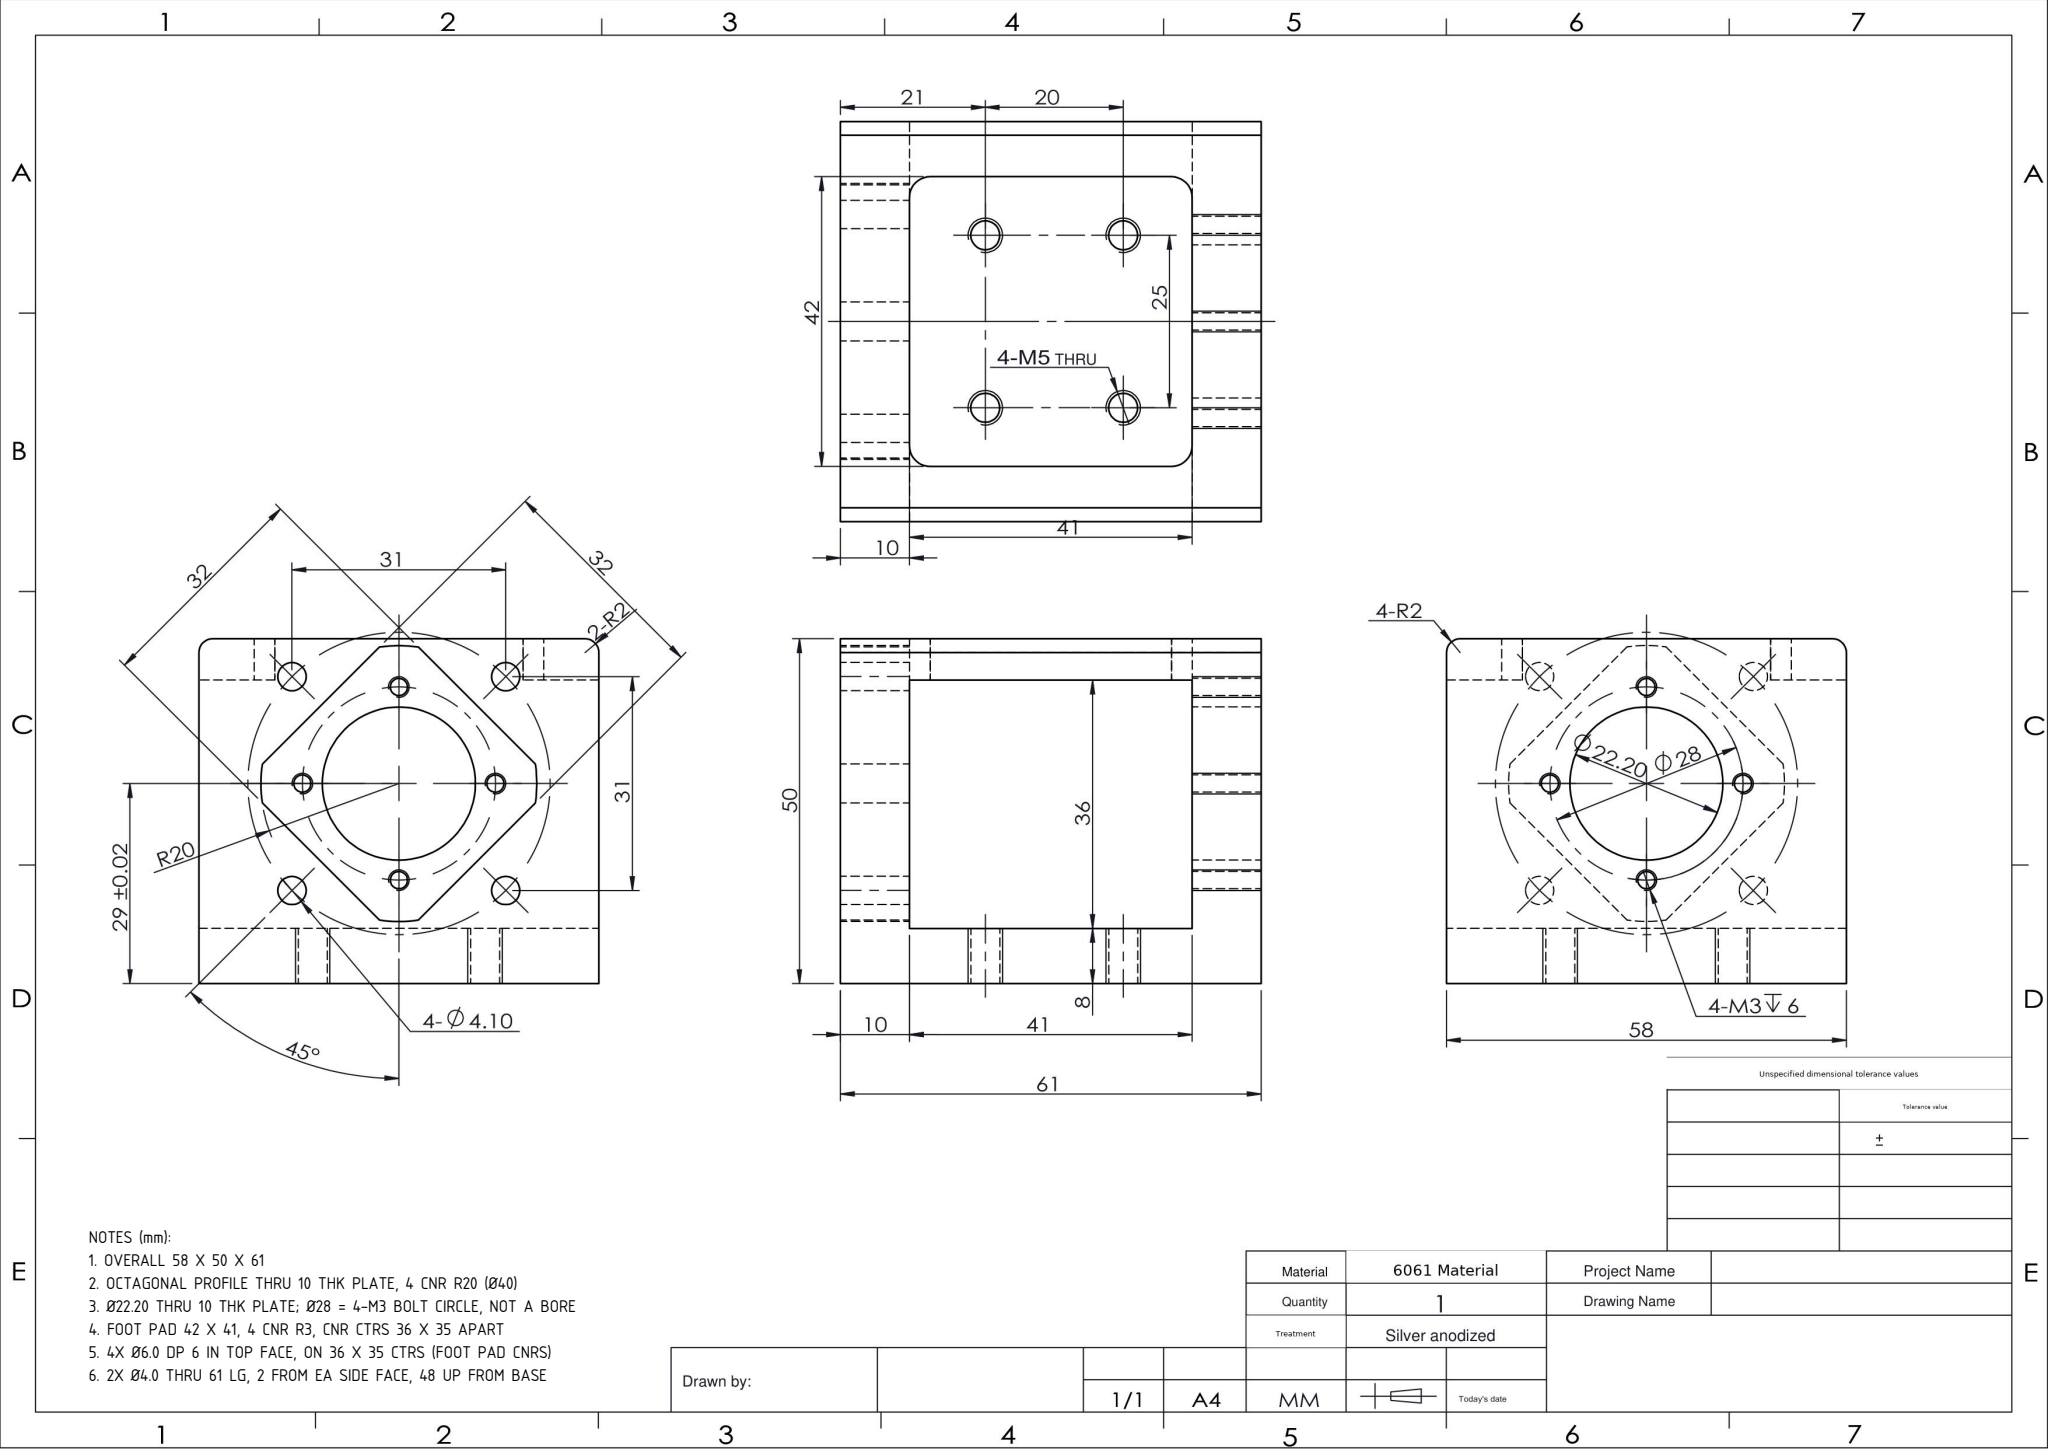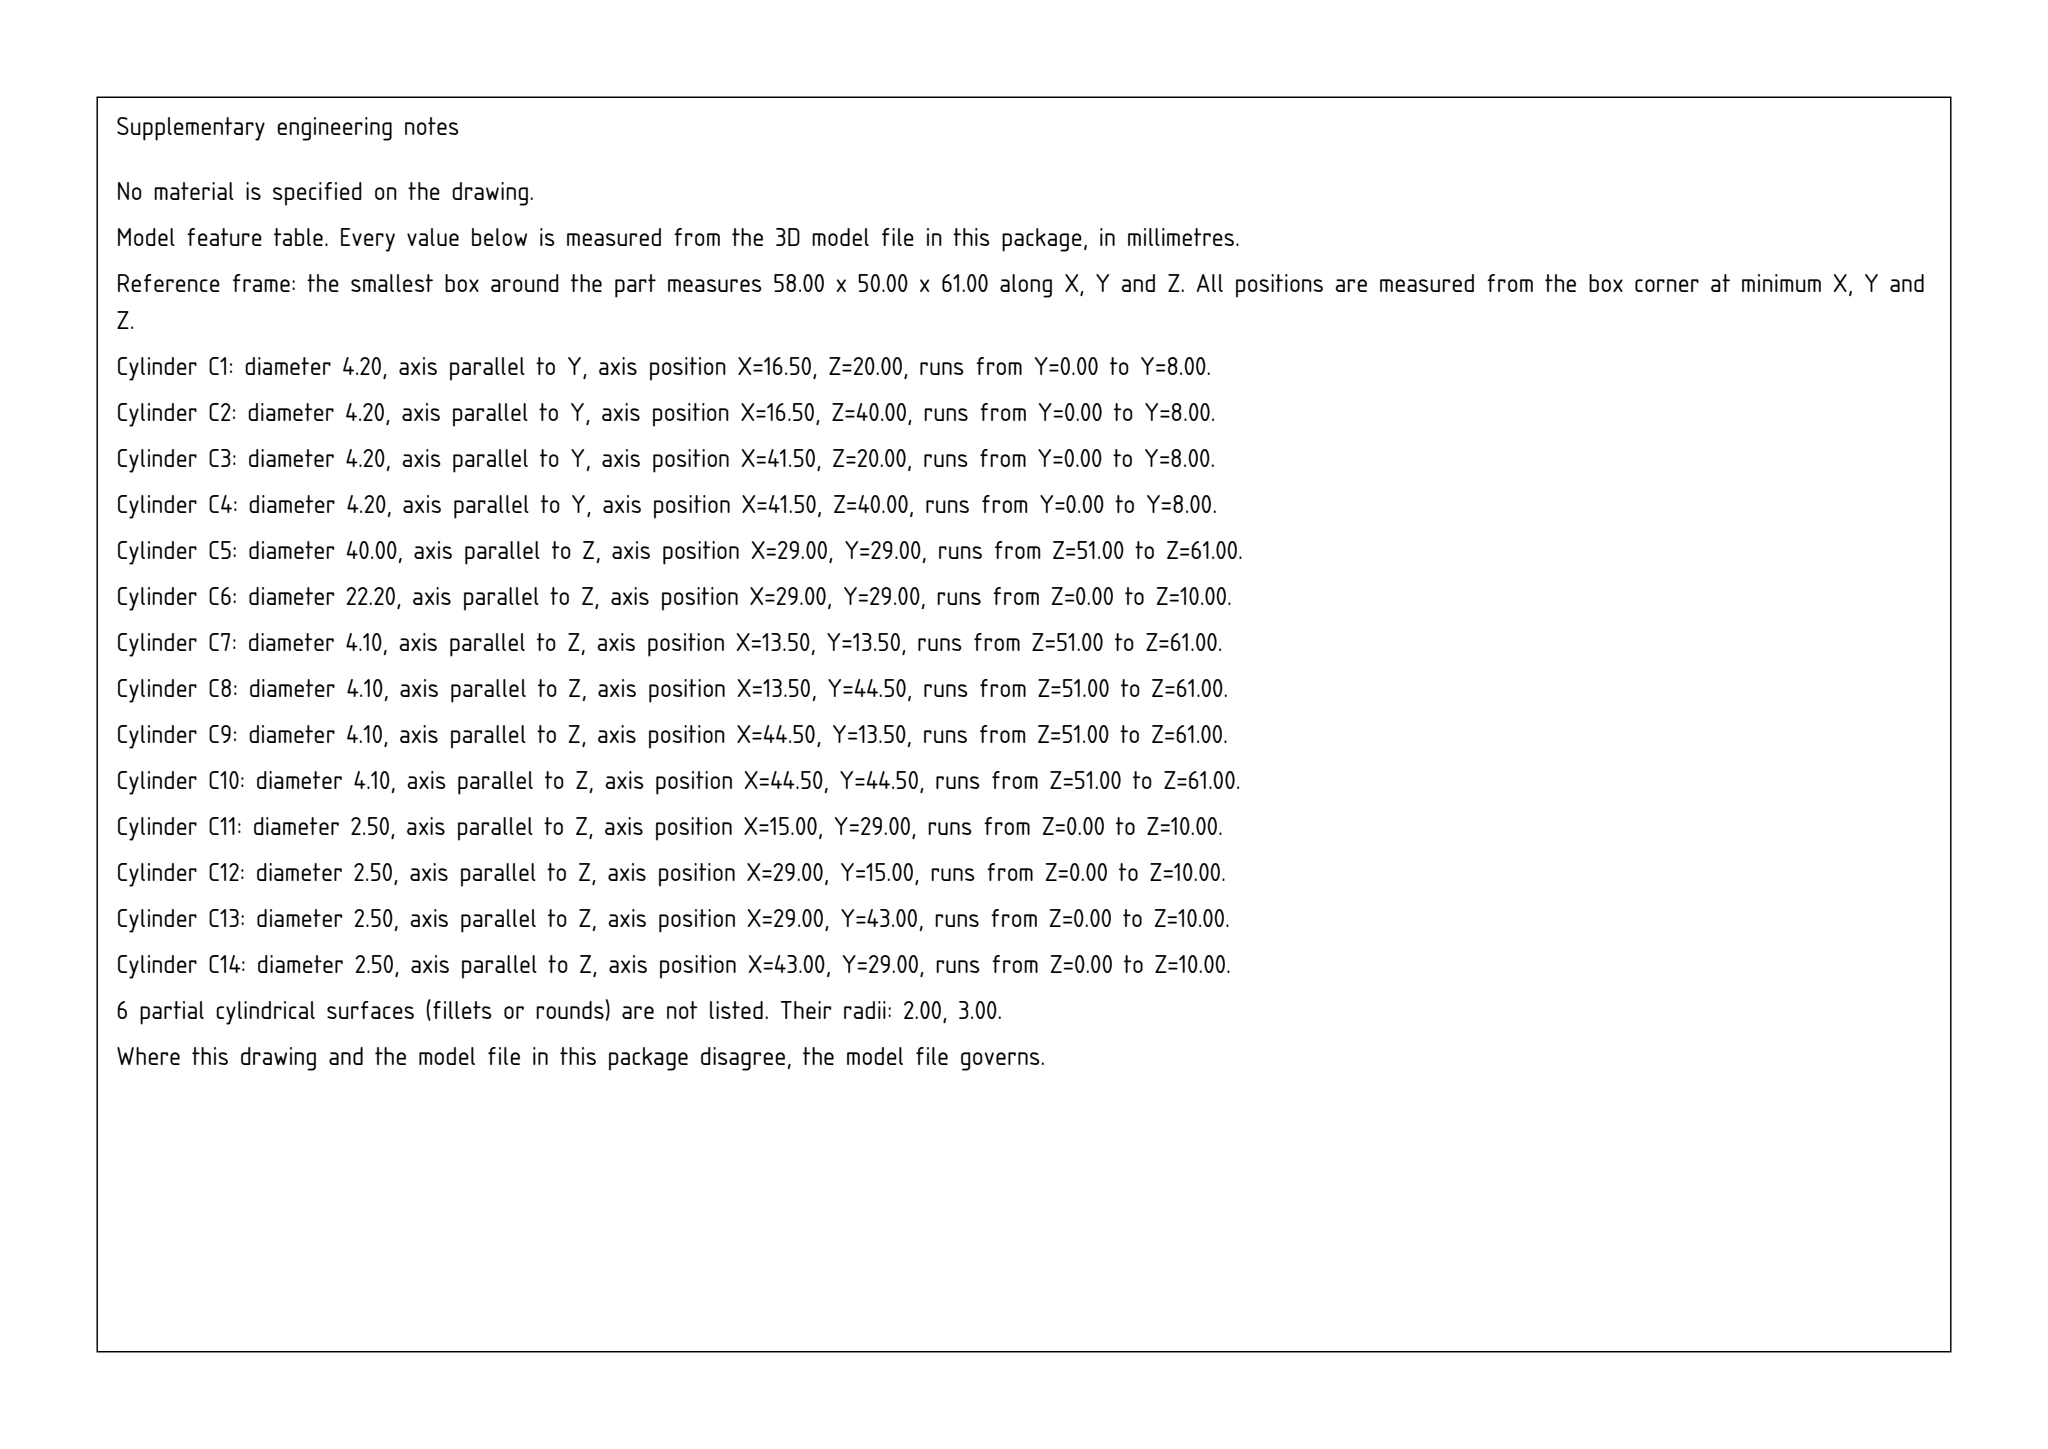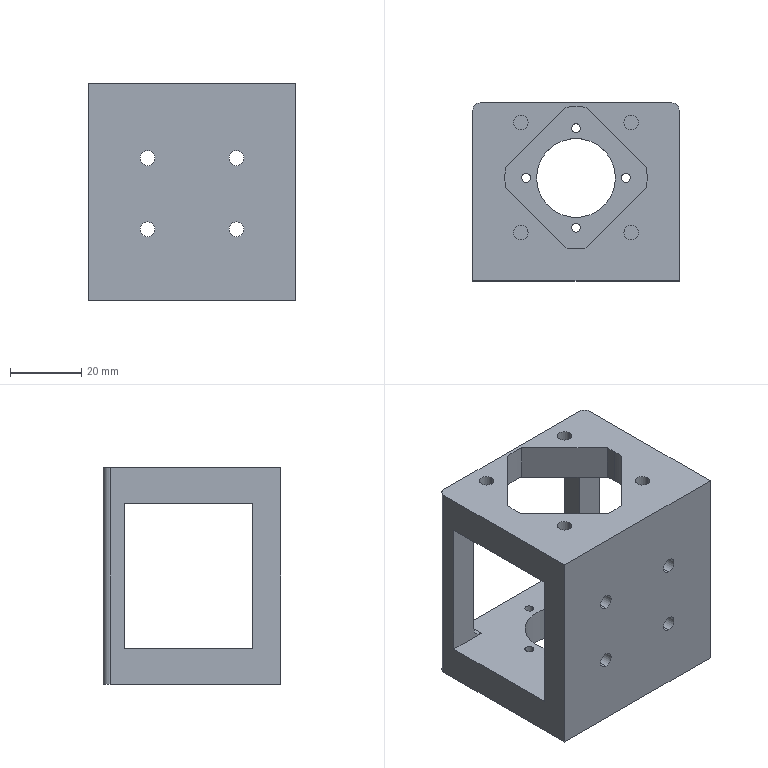Part | SolidWorks | mm | 1 solid | 54 faces | box 58 x 50 x 61 mm | volume 65913 mm3 | cylinder 37 | plane 17 | commonest cylinder face diameters 4.2 x8 2.5 x8 4.1 x8 40 x5 6 x4 22.2 x2 4 x2
Drawing notes:
OVERALL 58 X 50 X 61 | from the solid: bbox_xyz 58 x 50 x 61
OCTAGONAL PROFILE THRU 10 THK PLATE, 4 CNR R20 (Ø40) | from the solid: Ø40 (R20) faces axis Z at (29,29) len 10 = full plate thk; z planes only 0,10,51,61
Ø22.20 THRU 10 THK PLATE; Ø28 = 4-M3 BOLT CIRCLE, NOT A BORE | from the solid: Ø22.20 axis Z at (29,29) len 10; 4X Ø2.5 (M3) at R14 from CL = Ø28 BCD; no Ø28 cyl
FOOT PAD 42 X 41, 4 CNR R3, CNR CTRS 36 X 35 APART | from the solid: Ø6 y-axis cyls at (11,13)(11,48)(47,13)(47,48) = R3 cnrs; pad x8-50 (42), z10-51 (41)
4X Ø6.0 DP 6 IN TOP FACE, ON 36 X 35 CTRS (FOOT PAD CNRS) | from the solid: Ø6.0 axis y len 6 at (x,z)=(11,13),(11,48),(47,13),(47,48) from y=50 top face
2X Ø4.0 THRU 61 LG, 2 FROM EA SIDE FACE, 48 UP FROM BASE | from the solid: Ø4.0 axis z len 61 at (x,y)=(2,48) and (56,48); bbox 58 wide, base y=0
build123d program:
from build123d import *

# Parameters (mm, degrees)
SKETCH1_W                      = 58
SKETCH1_H                      = 50
BOSS_EXTRUDE1_DEPTH            = 61
M5_TAPPED_HOLE1_AT_2_COUNT     = 2
M5_TAPPED_HOLE1_AT_2_PITCH     = 25
SKETCH4_R                      = 11.1
CUT_EXTRUDE1_DEPTH             = 98.903
FILLET1_R                      = 2
F_4_1_4_1_DIAMETER_HOLE1_D     = 4.1
F_4_1_4_1_DIAMETER_HOLE1_DEPTH = 20
CIRPATTERN1_COUNT              = 4
CUT_EXTRUDE2_DEPTH             = 51
M3_TAPPED_HOLE2_D              = 2.5
CIRPATTERN2_COUNT              = 4
SKETCH10_W                     = 41
SKETCH10_H                     = 36
CUT_EXTRUDE3_DEPTH             = 98.903
SKETCH11_W                     = 42
SKETCH11_H                     = 41
CUT_EXTRUDE4_DEPTH             = 10
LPATTERN1_COUNT                = 2
LPATTERN1_PITCH                = 20
FILLET2_R                      = 3


with BuildPart() as part:
    # Sketch1 → Boss-Extrude1 (new body)
    with BuildSketch(Plane.XY):
        with Locations((29, 25)):
            Rectangle(SKETCH1_W, SKETCH1_H)
    extrude(amount=BOSS_EXTRUDE1_DEPTH)

    # Sketch2 → M5 Tapped Hole1 (revolve, cut)
    with BuildSketch(Plane(origin=(16.5, 0, 20), x_dir=(0, 0, -1), z_dir=(1, 0, 0))):
        Polygon((0, 0), (0, 13.662), (2.1, 12.4), (2.1, 0), align=None)
    m5_tapped_hole1 = revolve(axis=Axis((16.5, -6.35, 20), (0, 1, 0)), mode=Mode.SUBTRACT)

    # M5 Tapped Hole1 at 2: M5 Tapped Hole1 ×2
    with Locations(*[(i * M5_TAPPED_HOLE1_AT_2_PITCH, 0, 0) for i in range(1, M5_TAPPED_HOLE1_AT_2_COUNT)]):
        add(m5_tapped_hole1, mode=Mode.SUBTRACT)

    # Sketch4 → Cut-Extrude1 (cut, through all)
    with BuildSketch(Plane.XY.offset(61)):
        with Locations((29, 29)):
            Circle(SKETCH4_R)
    extrude(amount=-CUT_EXTRUDE1_DEPTH, mode=Mode.SUBTRACT)

    # Fillet1
    fillet1_edges = [part.edges().sort_by_distance(p)[0] for p in [
        (0, 50, 30.5),
        (58, 50, 30.5),
    ]]
    fillet(fillet1_edges, radius=FILLET1_R)

    # 4.1 _4.1_ Diameter Hole1
    with Locations(Plane.XY.offset(61)):
        with Locations((13.5, 44.5)):
            f_4_1_4_1_diameter_hole1 = Hole(F_4_1_4_1_DIAMETER_HOLE1_D / 2, depth=F_4_1_4_1_DIAMETER_HOLE1_DEPTH)

    # CirPattern1: 4.1 _4.1_ Diameter Hole1 ×4 about axis
    cirpattern1_axis = Axis((29, 29, 0), (0, 0, 1))
    for i in range(1, CIRPATTERN1_COUNT):
        add(f_4_1_4_1_diameter_hole1.rotate(cirpattern1_axis, i * 360 / CIRPATTERN1_COUNT), mode=Mode.SUBTRACT)

    # Sketch7 → Cut-Extrude2 (cut)
    with BuildSketch(Plane.XY.offset(61)):
        with BuildLine():
            Line((31.828, 48.799), (48.799, 31.828))
            ThreePointArc((48.799, 31.828), (49, 29), (48.799, 26.172))
            Line((48.799, 26.172), (31.828, 9.201))
            ThreePointArc((31.828, 9.201), (29, 9), (26.172, 9.201))
            Line((26.172, 9.201), (9.201, 26.172))
            ThreePointArc((9.201, 26.172), (9, 29), (9.201, 31.828))
            Line((9.201, 31.828), (26.172, 48.799))
            ThreePointArc((26.172, 48.799), (29, 49), (31.828, 48.799))
        make_face()
    extrude(amount=-CUT_EXTRUDE2_DEPTH, mode=Mode.SUBTRACT)

    # M3 Tapped Hole2 (through all)
    with Locations(Plane.XY.offset(10)):
        with Locations((29, 43)):
            m3_tapped_hole2 = Hole(M3_TAPPED_HOLE2_D / 2)

    # CirPattern2: M3 Tapped Hole2 ×4 about axis
    cirpattern2_axis = Axis((29, 29, 0), (0, 0, 1))
    for i in range(1, CIRPATTERN2_COUNT):
        add(m3_tapped_hole2.rotate(cirpattern2_axis, i * 360 / CIRPATTERN2_COUNT), mode=Mode.SUBTRACT)

    # Sketch10 → Cut-Extrude3 (cut, through all)
    with BuildSketch(Plane.ZY):
        with Locations((30.5, 26)):
            Rectangle(SKETCH10_W, SKETCH10_H)
    extrude(amount=-CUT_EXTRUDE3_DEPTH, mode=Mode.SUBTRACT)

    # Sketch11 → Cut-Extrude4 (cut)
    with BuildSketch(Plane(origin=(0, 50, 0), x_dir=(1, 0, 0), z_dir=(0, 1, 0))):
        with Locations((29, -30.5)):
            Rectangle(SKETCH11_W, SKETCH11_H)
    extrude(amount=-CUT_EXTRUDE4_DEPTH, mode=Mode.SUBTRACT)

    # LPattern1: M5 Tapped Hole1 ×2
    with Locations(*[(0, 0, i * LPATTERN1_PITCH) for i in range(1, LPATTERN1_COUNT)]):
        add(m5_tapped_hole1, mode=Mode.SUBTRACT)

    # LPattern1 copy 1 sketch → LPattern1 copy 1 (revolve, cut)
    with BuildSketch(Plane(origin=(41.5, 0, 40), x_dir=(0, 0, -1), z_dir=(1, 0, 0))):
        Polygon((0, 0), (0, 13.662), (2.1, 12.4), (2.1, 0), align=None)
    revolve(axis=Axis((41.5, -6.35, 40), (0, 1, 0)), mode=Mode.SUBTRACT)

    # Fillet2
    fillet2_edges = [part.edges().sort_by_distance(p)[0] for p in [
        (8, 47, 10),
        (50, 47, 51),
        (8, 47, 51),
        (50, 47, 10),
    ]]
    fillet(fillet2_edges, radius=FILLET2_R)


solid = part.part